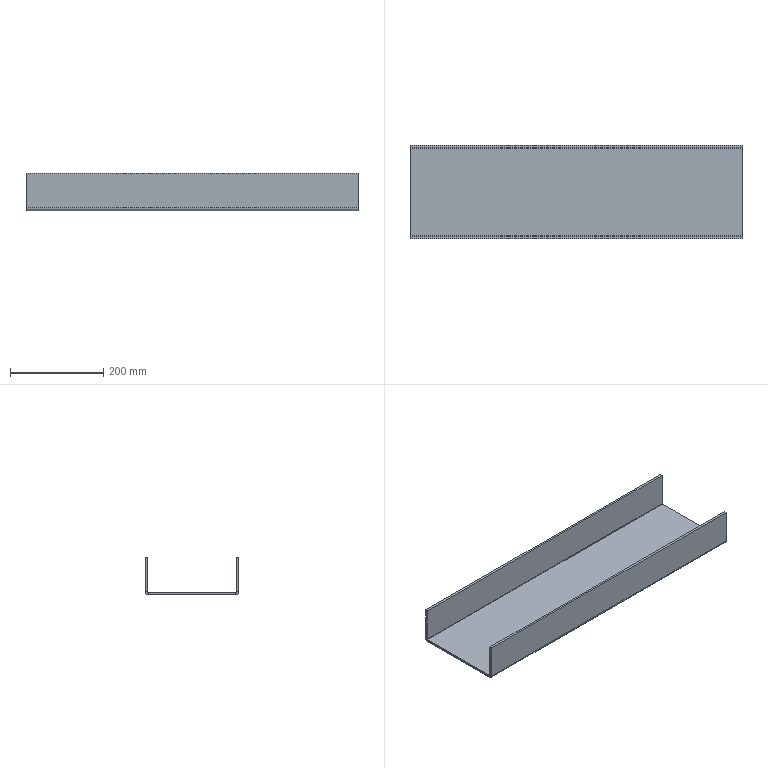Component | SolidWorks | ForkliftBasePlate-1 | 1 solid | 22 faces | box 712.5 x 200 x 80 mm | volume 1236977 mm3 | plane 18 | cylinder 4 | commonest cylinder face diameters 11.473 x2 1.473 x2 | material Q235
STEP:
#1=COLOUR_RGB('',0.7922,0.8196,0.9333);
#2=FILL_AREA_STYLE_COLOUR('',#1);
#3=FILL_AREA_STYLE('',(#2));
#4=SURFACE_STYLE_FILL_AREA(#3);
#5=SURFACE_SIDE_STYLE('',(#4));
#6=SURFACE_STYLE_USAGE(.BOTH.,#5);
#7=PRESENTATION_STYLE_ASSIGNMENT((#6));
#8=CARTESIAN_POINT('',(-18.136,36.701,107.705));
#9=VERTEX_POINT('',#8);
#10=CARTESIAN_POINT('',(-46.187,36.701,107.705));
#11=VERTEX_POINT('',#10);
#12=CARTESIAN_POINT('',(-18.136,36.701,107.705));
#13=DIRECTION('',(-1.,0.,0.));
#14=VECTOR('',#13,39.37);
#15=LINE('',#12,#14);
#16=EDGE_CURVE('',#9,#11,#15,.T.);
#17=ORIENTED_EDGE('',*,*,#16,.T.);
#18=CARTESIAN_POINT('',(-46.187,44.124,107.705));
#19=VERTEX_POINT('',#18);
#20=CARTESIAN_POINT('',(-46.187,44.349,107.705));
#21=DIRECTION('',(0.,-1.,0.));
#22=VECTOR('',#21,39.37);
#23=LINE('',#20,#22);
#24=EDGE_CURVE('',#19,#11,#23,.T.);
#25=ORIENTED_EDGE('',*,*,#24,.F.);
#26=CARTESIAN_POINT('',(-18.136,44.124,107.705));
#27=VERTEX_POINT('',#26);
#28=CARTESIAN_POINT('',(-46.187,44.124,107.705));
#29=DIRECTION('',(1.,0.,0.));
#30=VECTOR('',#29,39.37);
#31=LINE('',#28,#30);
#32=EDGE_CURVE('',#19,#27,#31,.T.);
#33=ORIENTED_EDGE('',*,*,#32,.T.);
#34=CARTESIAN_POINT('',(-18.136,44.349,107.705));
#35=DIRECTION('',(0.,1.,0.));
#36=VECTOR('',#35,39.37);
#37=LINE('',#34,#36);
#38=EDGE_CURVE('',#9,#27,#37,.T.);
#39=ORIENTED_EDGE('',*,*,#38,.F.);
#40=EDGE_LOOP('',(#17,#25,#33,#39));
#41=FACE_OUTER_BOUND('',#40,.T.);
#42=CARTESIAN_POINT('',(-32.162,40.412,107.705));
#43=DIRECTION('',(0.,0.,1.));
#44=DIRECTION('',(1.,0.,0.));
#45=AXIS2_PLACEMENT_3D('',#42,#43,#44);
#46=PLANE('',#45);
#47=ADVANCED_FACE('',(#41),#46,.F.);
#48=CARTESIAN_POINT('',(-46.187,44.124,107.902));
#49=VERTEX_POINT('',#48);
#50=CARTESIAN_POINT('',(-46.187,36.701,107.902));
#51=VERTEX_POINT('',#50);
#52=CARTESIAN_POINT('',(-46.187,44.349,107.902));
#53=DIRECTION('',(0.,-1.,0.));
#54=VECTOR('',#53,39.37);
#55=LINE('',#52,#54);
#56=EDGE_CURVE('',#49,#51,#55,.T.);
#57=ORIENTED_EDGE('',*,*,#56,.T.);
#58=CARTESIAN_POINT('',(-18.136,36.701,107.902));
#59=VERTEX_POINT('',#58);
#60=CARTESIAN_POINT('',(-18.136,36.701,107.902));
#61=DIRECTION('',(-1.,0.,0.));
#62=VECTOR('',#61,39.37);
#63=LINE('',#60,#62);
#64=EDGE_CURVE('',#59,#51,#63,.T.);
#65=ORIENTED_EDGE('',*,*,#64,.F.);
#66=CARTESIAN_POINT('',(-18.136,44.124,107.902));
#67=VERTEX_POINT('',#66);
#68=CARTESIAN_POINT('',(-18.136,44.349,107.902));
#69=DIRECTION('',(0.,1.,0.));
#70=VECTOR('',#69,39.37);
#71=LINE('',#68,#70);
#72=EDGE_CURVE('',#59,#67,#71,.T.);
#73=ORIENTED_EDGE('',*,*,#72,.T.);
#74=CARTESIAN_POINT('',(-46.187,44.124,107.902));
#75=DIRECTION('',(1.,0.,0.));
#76=VECTOR('',#75,39.37);
#77=LINE('',#74,#76);
#78=EDGE_CURVE('',#49,#67,#77,.T.);
#79=ORIENTED_EDGE('',*,*,#78,.F.);
#80=EDGE_LOOP('',(#57,#65,#73,#79));
#81=FACE_OUTER_BOUND('',#80,.T.);
#82=CARTESIAN_POINT('',(-32.162,40.412,107.902));
#83=DIRECTION('',(0.,0.,1.));
#84=DIRECTION('',(1.,0.,0.));
#85=AXIS2_PLACEMENT_3D('',#82,#83,#84);
#86=PLANE('',#85);
#87=ADVANCED_FACE('',(#81),#86,.T.);
#88=ORIENTED_EDGE('',*,*,#72,.F.);
#89=CARTESIAN_POINT('',(-18.136,36.701,107.902));
#90=DIRECTION('',(0.,0.,-1.));
#91=VECTOR('',#90,39.37);
#92=LINE('',#89,#91);
#93=EDGE_CURVE('',#59,#9,#92,.T.);
#94=ORIENTED_EDGE('',*,*,#93,.T.);
#95=ORIENTED_EDGE('',*,*,#38,.T.);
#96=CARTESIAN_POINT('',(-18.136,44.124,107.902));
#97=DIRECTION('',(0.,0.,-1.));
#98=VECTOR('',#97,39.37);
#99=LINE('',#96,#98);
#100=EDGE_CURVE('',#67,#27,#99,.T.);
#101=ORIENTED_EDGE('',*,*,#100,.F.);
#102=EDGE_LOOP('',(#88,#94,#95,#101));
#103=FACE_OUTER_BOUND('',#102,.T.);
#104=CARTESIAN_POINT('',(-18.136,44.349,107.705));
#105=DIRECTION('',(1.,0.,0.));
#106=DIRECTION('',(0.,0.,-1.));
#107=AXIS2_PLACEMENT_3D('',#104,#105,#106);
#108=PLANE('',#107);
#109=ADVANCED_FACE('',(#103),#108,.T.);
#110=CARTESIAN_POINT('',(-46.187,36.701,107.902));
#111=DIRECTION('',(0.,0.,-1.));
#112=VECTOR('',#111,39.37);
#113=LINE('',#110,#112);
#114=EDGE_CURVE('',#51,#11,#113,.T.);
#115=ORIENTED_EDGE('',*,*,#114,.F.);
#116=ORIENTED_EDGE('',*,*,#56,.F.);
#117=CARTESIAN_POINT('',(-46.187,44.124,107.902));
#118=DIRECTION('',(0.,0.,-1.));
#119=VECTOR('',#118,39.37);
#120=LINE('',#117,#119);
#121=EDGE_CURVE('',#49,#19,#120,.T.);
#122=ORIENTED_EDGE('',*,*,#121,.T.);
#123=ORIENTED_EDGE('',*,*,#24,.T.);
#124=EDGE_LOOP('',(#115,#116,#122,#123));
#125=FACE_OUTER_BOUND('',#124,.T.);
#126=CARTESIAN_POINT('',(-46.187,44.349,107.705));
#127=DIRECTION('',(-1.,0.,0.));
#128=DIRECTION('',(0.,0.,1.));
#129=AXIS2_PLACEMENT_3D('',#126,#127,#128);
#130=PLANE('',#129);
#131=ADVANCED_FACE('',(#125),#130,.T.);
#132=CARTESIAN_POINT('',(-18.136,44.153,107.931));
#133=VERTEX_POINT('',#132);
#134=CARTESIAN_POINT('',(-18.136,44.349,107.931));
#135=VERTEX_POINT('',#134);
#136=CARTESIAN_POINT('',(-18.136,44.349,107.931));
#137=DIRECTION('',(0.,1.,-0.));
#138=VECTOR('',#137,39.37);
#139=LINE('',#136,#138);
#140=EDGE_CURVE('',#133,#135,#139,.T.);
#141=ORIENTED_EDGE('',*,*,#140,.F.);
#142=CARTESIAN_POINT('',(-18.136,44.124,107.931));
#143=DIRECTION('',(1.,0.,0.));
#144=DIRECTION('',(0.,0.,1.));
#145=AXIS2_PLACEMENT_3D('',#142,#143,#144);
#146=CIRCLE('',#145,0.029);
#147=EDGE_CURVE('',#67,#133,#146,.T.);
#148=ORIENTED_EDGE('',*,*,#147,.F.);
#149=ORIENTED_EDGE('',*,*,#100,.T.);
#150=CARTESIAN_POINT('',(-18.136,44.124,107.931));
#151=DIRECTION('',(1.,0.,0.));
#152=DIRECTION('',(0.,0.,1.));
#153=AXIS2_PLACEMENT_3D('',#150,#151,#152);
#154=CIRCLE('',#153,0.2259);
#155=EDGE_CURVE('',#27,#135,#154,.T.);
#156=ORIENTED_EDGE('',*,*,#155,.T.);
#157=EDGE_LOOP('',(#141,#148,#149,#156));
#158=FACE_OUTER_BOUND('',#157,.T.);
#159=CARTESIAN_POINT('',(-18.136,44.124,107.931));
#160=DIRECTION('',(1.,0.,0.));
#161=DIRECTION('',(0.,0.,-1.));
#162=AXIS2_PLACEMENT_3D('',#159,#160,#161);
#163=PLANE('',#162);
#164=ADVANCED_FACE('',(#158),#163,.T.);
#165=CARTESIAN_POINT('',(-46.187,44.153,107.931));
#166=VERTEX_POINT('',#165);
#167=CARTESIAN_POINT('',(-46.187,44.124,107.931));
#168=DIRECTION('',(-1.,0.,0.));
#169=DIRECTION('',(0.,0.,1.));
#170=AXIS2_PLACEMENT_3D('',#167,#168,#169);
#171=CIRCLE('',#170,0.029);
#172=EDGE_CURVE('',#166,#49,#171,.T.);
#173=ORIENTED_EDGE('',*,*,#172,.F.);
#174=CARTESIAN_POINT('',(-46.187,44.349,107.931));
#175=VERTEX_POINT('',#174);
#176=CARTESIAN_POINT('',(-46.187,44.153,107.931));
#177=DIRECTION('',(0.,1.,-0.));
#178=VECTOR('',#177,39.37);
#179=LINE('',#176,#178);
#180=EDGE_CURVE('',#166,#175,#179,.T.);
#181=ORIENTED_EDGE('',*,*,#180,.T.);
#182=CARTESIAN_POINT('',(-46.187,44.124,107.931));
#183=DIRECTION('',(-1.,0.,0.));
#184=DIRECTION('',(0.,0.,1.));
#185=AXIS2_PLACEMENT_3D('',#182,#183,#184);
#186=CIRCLE('',#185,0.2259);
#187=EDGE_CURVE('',#175,#19,#186,.T.);
#188=ORIENTED_EDGE('',*,*,#187,.T.);
#189=ORIENTED_EDGE('',*,*,#121,.F.);
#190=EDGE_LOOP('',(#173,#181,#188,#189));
#191=FACE_OUTER_BOUND('',#190,.T.);
#192=CARTESIAN_POINT('',(-46.187,44.124,107.931));
#193=DIRECTION('',(1.,0.,0.));
#194=DIRECTION('',(0.,0.,-1.));
#195=AXIS2_PLACEMENT_3D('',#192,#193,#194);
#196=PLANE('',#195);
#197=ADVANCED_FACE('',(#191),#196,.F.);
#198=ORIENTED_EDGE('',*,*,#32,.F.);
#199=ORIENTED_EDGE('',*,*,#187,.F.);
#200=CARTESIAN_POINT('',(-32.162,44.349,107.931));
#201=DIRECTION('',(-1.,-0.,-0.));
#202=VECTOR('',#201,39.37);
#203=LINE('',#200,#202);
#204=EDGE_CURVE('',#135,#175,#203,.T.);
#205=ORIENTED_EDGE('',*,*,#204,.F.);
#206=ORIENTED_EDGE('',*,*,#155,.F.);
#207=EDGE_LOOP('',(#198,#199,#205,#206));
#208=FACE_OUTER_BOUND('',#207,.T.);
#209=CARTESIAN_POINT('',(-46.187,44.124,107.931));
#210=DIRECTION('',(-1.,0.,0.));
#211=DIRECTION('',(0.,1.,0.));
#212=AXIS2_PLACEMENT_3D('',#209,#210,#211);
#213=CYLINDRICAL_SURFACE('',#212,0.2259);
#214=ADVANCED_FACE('',(#208),#213,.T.);
#215=ORIENTED_EDGE('',*,*,#78,.T.);
#216=ORIENTED_EDGE('',*,*,#147,.T.);
#217=CARTESIAN_POINT('',(-18.136,44.153,107.931));
#218=DIRECTION('',(-1.,-0.,-0.));
#219=VECTOR('',#218,39.37);
#220=LINE('',#217,#219);
#221=EDGE_CURVE('',#133,#166,#220,.T.);
#222=ORIENTED_EDGE('',*,*,#221,.T.);
#223=ORIENTED_EDGE('',*,*,#172,.T.);
#224=EDGE_LOOP('',(#215,#216,#222,#223));
#225=FACE_OUTER_BOUND('',#224,.T.);
#226=CARTESIAN_POINT('',(-46.187,44.124,107.931));
#227=DIRECTION('',(-1.,0.,0.));
#228=DIRECTION('',(0.,1.,0.));
#229=AXIS2_PLACEMENT_3D('',#226,#227,#228);
#230=CYLINDRICAL_SURFACE('',#229,0.029);
#231=ADVANCED_FACE('',(#225),#230,.F.);
#232=CARTESIAN_POINT('',(-46.187,44.349,110.855));
#233=VERTEX_POINT('',#232);
#234=CARTESIAN_POINT('',(-46.187,44.349,107.902));
#235=DIRECTION('',(0.,-0.,-1.));
#236=VECTOR('',#235,39.37);
#237=LINE('',#234,#236);
#238=EDGE_CURVE('',#233,#175,#237,.T.);
#239=ORIENTED_EDGE('',*,*,#238,.T.);
#240=ORIENTED_EDGE('',*,*,#180,.F.);
#241=CARTESIAN_POINT('',(-46.187,44.153,110.855));
#242=VERTEX_POINT('',#241);
#243=CARTESIAN_POINT('',(-46.187,44.153,107.902));
#244=DIRECTION('',(0.,-0.,-1.));
#245=VECTOR('',#244,39.37);
#246=LINE('',#243,#245);
#247=EDGE_CURVE('',#242,#166,#246,.T.);
#248=ORIENTED_EDGE('',*,*,#247,.F.);
#249=CARTESIAN_POINT('',(-46.187,44.349,110.855));
#250=DIRECTION('',(0.,-1.,0.));
#251=VECTOR('',#250,39.37);
#252=LINE('',#249,#251);
#253=EDGE_CURVE('',#233,#242,#252,.T.);
#254=ORIENTED_EDGE('',*,*,#253,.F.);
#255=EDGE_LOOP('',(#239,#240,#248,#254));
#256=FACE_OUTER_BOUND('',#255,.T.);
#257=CARTESIAN_POINT('',(-46.187,44.349,107.902));
#258=DIRECTION('',(-1.,0.,0.));
#259=DIRECTION('',(0.,0.,1.));
#260=AXIS2_PLACEMENT_3D('',#257,#258,#259);
#261=PLANE('',#260);
#262=ADVANCED_FACE('',(#256),#261,.T.);
#263=CARTESIAN_POINT('',(-18.136,44.153,110.855));
#264=VERTEX_POINT('',#263);
#265=CARTESIAN_POINT('',(-18.136,44.153,107.902));
#266=DIRECTION('',(0.,0.,1.));
#267=VECTOR('',#266,39.37);
#268=LINE('',#265,#267);
#269=EDGE_CURVE('',#133,#264,#268,.T.);
#270=ORIENTED_EDGE('',*,*,#269,.F.);
#271=ORIENTED_EDGE('',*,*,#140,.T.);
#272=CARTESIAN_POINT('',(-18.136,44.349,110.855));
#273=VERTEX_POINT('',#272);
#274=CARTESIAN_POINT('',(-18.136,44.349,110.855));
#275=DIRECTION('',(0.,0.,1.));
#276=VECTOR('',#275,39.37);
#277=LINE('',#274,#276);
#278=EDGE_CURVE('',#135,#273,#277,.T.);
#279=ORIENTED_EDGE('',*,*,#278,.T.);
#280=CARTESIAN_POINT('',(-18.136,44.349,110.855));
#281=DIRECTION('',(0.,-1.,0.));
#282=VECTOR('',#281,39.37);
#283=LINE('',#280,#282);
#284=EDGE_CURVE('',#273,#264,#283,.T.);
#285=ORIENTED_EDGE('',*,*,#284,.T.);
#286=EDGE_LOOP('',(#270,#271,#279,#285));
#287=FACE_OUTER_BOUND('',#286,.T.);
#288=CARTESIAN_POINT('',(-18.136,44.349,110.855));
#289=DIRECTION('',(1.,0.,0.));
#290=DIRECTION('',(0.,0.,-1.));
#291=AXIS2_PLACEMENT_3D('',#288,#289,#290);
#292=PLANE('',#291);
#293=ADVANCED_FACE('',(#287),#292,.T.);
#294=ORIENTED_EDGE('',*,*,#278,.F.);
#295=ORIENTED_EDGE('',*,*,#204,.T.);
#296=ORIENTED_EDGE('',*,*,#238,.F.);
#297=CARTESIAN_POINT('',(-46.187,44.349,110.855));
#298=DIRECTION('',(-1.,0.,0.));
#299=VECTOR('',#298,39.37);
#300=LINE('',#297,#299);
#301=EDGE_CURVE('',#273,#233,#300,.T.);
#302=ORIENTED_EDGE('',*,*,#301,.F.);
#303=EDGE_LOOP('',(#294,#295,#296,#302));
#304=FACE_OUTER_BOUND('',#303,.T.);
#305=CARTESIAN_POINT('',(-32.162,44.349,107.902));
#306=DIRECTION('',(0.,1.,-0.));
#307=DIRECTION('',(0.,0.,1.));
#308=AXIS2_PLACEMENT_3D('',#305,#306,#307);
#309=PLANE('',#308);
#310=ADVANCED_FACE('',(#304),#309,.T.);
#311=ORIENTED_EDGE('',*,*,#221,.F.);
#312=ORIENTED_EDGE('',*,*,#269,.T.);
#313=CARTESIAN_POINT('',(-32.162,44.153,110.855));
#314=DIRECTION('',(-1.,0.,0.));
#315=VECTOR('',#314,39.37);
#316=LINE('',#313,#315);
#317=EDGE_CURVE('',#264,#242,#316,.T.);
#318=ORIENTED_EDGE('',*,*,#317,.T.);
#319=ORIENTED_EDGE('',*,*,#247,.T.);
#320=EDGE_LOOP('',(#311,#312,#318,#319));
#321=FACE_OUTER_BOUND('',#320,.T.);
#322=CARTESIAN_POINT('',(-32.162,44.153,107.902));
#323=DIRECTION('',(0.,1.,-0.));
#324=DIRECTION('',(0.,0.,1.));
#325=AXIS2_PLACEMENT_3D('',#322,#323,#324);
#326=PLANE('',#325);
#327=ADVANCED_FACE('',(#321),#326,.F.);
#328=ORIENTED_EDGE('',*,*,#317,.F.);
#329=ORIENTED_EDGE('',*,*,#284,.F.);
#330=ORIENTED_EDGE('',*,*,#301,.T.);
#331=ORIENTED_EDGE('',*,*,#253,.T.);
#332=EDGE_LOOP('',(#328,#329,#330,#331));
#333=FACE_OUTER_BOUND('',#332,.T.);
#334=CARTESIAN_POINT('',(-46.187,44.349,110.855));
#335=DIRECTION('',(0.,0.,1.));
#336=DIRECTION('',(0.,-1.,0.));
#337=AXIS2_PLACEMENT_3D('',#334,#335,#336);
#338=PLANE('',#337);
#339=ADVANCED_FACE('',(#333),#338,.T.);
#340=CARTESIAN_POINT('',(-46.187,36.672,107.931));
#341=VERTEX_POINT('',#340);
#342=CARTESIAN_POINT('',(-46.187,36.475,107.931));
#343=VERTEX_POINT('',#342);
#344=CARTESIAN_POINT('',(-46.187,36.475,107.931));
#345=DIRECTION('',(0.,-1.,-0.));
#346=VECTOR('',#345,39.37);
#347=LINE('',#344,#346);
#348=EDGE_CURVE('',#341,#343,#347,.T.);
#349=ORIENTED_EDGE('',*,*,#348,.F.);
#350=CARTESIAN_POINT('',(-46.187,36.701,107.931));
#351=DIRECTION('',(-1.,0.,0.));
#352=DIRECTION('',(0.,0.,-1.));
#353=AXIS2_PLACEMENT_3D('',#350,#351,#352);
#354=CIRCLE('',#353,0.029);
#355=EDGE_CURVE('',#51,#341,#354,.T.);
#356=ORIENTED_EDGE('',*,*,#355,.F.);
#357=ORIENTED_EDGE('',*,*,#114,.T.);
#358=CARTESIAN_POINT('',(-46.187,36.701,107.931));
#359=DIRECTION('',(-1.,0.,0.));
#360=DIRECTION('',(0.,0.,-1.));
#361=AXIS2_PLACEMENT_3D('',#358,#359,#360);
#362=CIRCLE('',#361,0.2259);
#363=EDGE_CURVE('',#11,#343,#362,.T.);
#364=ORIENTED_EDGE('',*,*,#363,.T.);
#365=EDGE_LOOP('',(#349,#356,#357,#364));
#366=FACE_OUTER_BOUND('',#365,.T.);
#367=CARTESIAN_POINT('',(-46.187,36.701,107.931));
#368=DIRECTION('',(-1.,0.,0.));
#369=DIRECTION('',(0.,0.,1.));
#370=AXIS2_PLACEMENT_3D('',#367,#368,#369);
#371=PLANE('',#370);
#372=ADVANCED_FACE('',(#366),#371,.T.);
#373=CARTESIAN_POINT('',(-18.136,36.672,107.931));
#374=VERTEX_POINT('',#373);
#375=CARTESIAN_POINT('',(-18.136,36.701,107.931));
#376=DIRECTION('',(1.,0.,0.));
#377=DIRECTION('',(0.,0.,-1.));
#378=AXIS2_PLACEMENT_3D('',#375,#376,#377);
#379=CIRCLE('',#378,0.029);
#380=EDGE_CURVE('',#374,#59,#379,.T.);
#381=ORIENTED_EDGE('',*,*,#380,.F.);
#382=CARTESIAN_POINT('',(-18.136,36.475,107.931));
#383=VERTEX_POINT('',#382);
#384=CARTESIAN_POINT('',(-18.136,36.672,107.931));
#385=DIRECTION('',(0.,-1.,-0.));
#386=VECTOR('',#385,39.37);
#387=LINE('',#384,#386);
#388=EDGE_CURVE('',#374,#383,#387,.T.);
#389=ORIENTED_EDGE('',*,*,#388,.T.);
#390=CARTESIAN_POINT('',(-18.136,36.701,107.931));
#391=DIRECTION('',(1.,0.,0.));
#392=DIRECTION('',(0.,0.,-1.));
#393=AXIS2_PLACEMENT_3D('',#390,#391,#392);
#394=CIRCLE('',#393,0.2259);
#395=EDGE_CURVE('',#383,#9,#394,.T.);
#396=ORIENTED_EDGE('',*,*,#395,.T.);
#397=ORIENTED_EDGE('',*,*,#93,.F.);
#398=EDGE_LOOP('',(#381,#389,#396,#397));
#399=FACE_OUTER_BOUND('',#398,.T.);
#400=CARTESIAN_POINT('',(-18.136,36.701,107.931));
#401=DIRECTION('',(-1.,0.,0.));
#402=DIRECTION('',(0.,0.,1.));
#403=AXIS2_PLACEMENT_3D('',#400,#401,#402);
#404=PLANE('',#403);
#405=ADVANCED_FACE('',(#399),#404,.F.);
#406=ORIENTED_EDGE('',*,*,#16,.F.);
#407=ORIENTED_EDGE('',*,*,#395,.F.);
#408=CARTESIAN_POINT('',(-32.162,36.475,107.931));
#409=DIRECTION('',(1.,-0.,0.));
#410=VECTOR('',#409,39.37);
#411=LINE('',#408,#410);
#412=EDGE_CURVE('',#343,#383,#411,.T.);
#413=ORIENTED_EDGE('',*,*,#412,.F.);
#414=ORIENTED_EDGE('',*,*,#363,.F.);
#415=EDGE_LOOP('',(#406,#407,#413,#414));
#416=FACE_OUTER_BOUND('',#415,.T.);
#417=CARTESIAN_POINT('',(-18.136,36.701,107.931));
#418=DIRECTION('',(1.,0.,0.));
#419=DIRECTION('',(0.,-1.,0.));
#420=AXIS2_PLACEMENT_3D('',#417,#418,#419);
#421=CYLINDRICAL_SURFACE('',#420,0.2259);
#422=ADVANCED_FACE('',(#416),#421,.T.);
#423=ORIENTED_EDGE('',*,*,#64,.T.);
#424=ORIENTED_EDGE('',*,*,#355,.T.);
#425=CARTESIAN_POINT('',(-46.187,36.672,107.931));
#426=DIRECTION('',(1.,-0.,0.));
#427=VECTOR('',#426,39.37);
#428=LINE('',#425,#427);
#429=EDGE_CURVE('',#341,#374,#428,.T.);
#430=ORIENTED_EDGE('',*,*,#429,.T.);
#431=ORIENTED_EDGE('',*,*,#380,.T.);
#432=EDGE_LOOP('',(#423,#424,#430,#431));
#433=FACE_OUTER_BOUND('',#432,.T.);
#434=CARTESIAN_POINT('',(-18.136,36.701,107.931));
#435=DIRECTION('',(1.,0.,0.));
#436=DIRECTION('',(0.,-1.,0.));
#437=AXIS2_PLACEMENT_3D('',#434,#435,#436);
#438=CYLINDRICAL_SURFACE('',#437,0.029);
#439=ADVANCED_FACE('',(#433),#438,.F.);
#440=CARTESIAN_POINT('',(-18.136,36.475,110.855));
#441=VERTEX_POINT('',#440);
#442=CARTESIAN_POINT('',(-18.136,36.475,107.902));
#443=DIRECTION('',(0.,0.,-1.));
#444=VECTOR('',#443,39.37);
#445=LINE('',#442,#444);
#446=EDGE_CURVE('',#441,#383,#445,.T.);
#447=ORIENTED_EDGE('',*,*,#446,.T.);
#448=ORIENTED_EDGE('',*,*,#388,.F.);
#449=CARTESIAN_POINT('',(-18.136,36.672,110.855));
#450=VERTEX_POINT('',#449);
#451=CARTESIAN_POINT('',(-18.136,36.672,107.902));
#452=DIRECTION('',(0.,0.,-1.));
#453=VECTOR('',#452,39.37);
#454=LINE('',#451,#453);
#455=EDGE_CURVE('',#450,#374,#454,.T.);
#456=ORIENTED_EDGE('',*,*,#455,.F.);
#457=CARTESIAN_POINT('',(-18.136,36.475,110.855));
#458=DIRECTION('',(0.,1.,0.));
#459=VECTOR('',#458,39.37);
#460=LINE('',#457,#459);
#461=EDGE_CURVE('',#441,#450,#460,.T.);
#462=ORIENTED_EDGE('',*,*,#461,.F.);
#463=EDGE_LOOP('',(#447,#448,#456,#462));
#464=FACE_OUTER_BOUND('',#463,.T.);
#465=CARTESIAN_POINT('',(-18.136,36.475,107.902));
#466=DIRECTION('',(1.,0.,0.));
#467=DIRECTION('',(0.,0.,-1.));
#468=AXIS2_PLACEMENT_3D('',#465,#466,#467);
#469=PLANE('',#468);
#470=ADVANCED_FACE('',(#464),#469,.T.);
#471=CARTESIAN_POINT('',(-46.187,36.672,110.855));
#472=VERTEX_POINT('',#471);
#473=CARTESIAN_POINT('',(-46.187,36.672,107.902));
#474=DIRECTION('',(0.,-0.,1.));
#475=VECTOR('',#474,39.37);
#476=LINE('',#473,#475);
#477=EDGE_CURVE('',#341,#472,#476,.T.);
#478=ORIENTED_EDGE('',*,*,#477,.F.);
#479=ORIENTED_EDGE('',*,*,#348,.T.);
#480=CARTESIAN_POINT('',(-46.187,36.475,110.855));
#481=VERTEX_POINT('',#480);
#482=CARTESIAN_POINT('',(-46.187,36.475,110.855));
#483=DIRECTION('',(0.,-0.,1.));
#484=VECTOR('',#483,39.37);
#485=LINE('',#482,#484);
#486=EDGE_CURVE('',#343,#481,#485,.T.);
#487=ORIENTED_EDGE('',*,*,#486,.T.);
#488=CARTESIAN_POINT('',(-46.187,36.475,110.855));
#489=DIRECTION('',(0.,1.,0.));
#490=VECTOR('',#489,39.37);
#491=LINE('',#488,#490);
#492=EDGE_CURVE('',#481,#472,#491,.T.);
#493=ORIENTED_EDGE('',*,*,#492,.T.);
#494=EDGE_LOOP('',(#478,#479,#487,#493));
#495=FACE_OUTER_BOUND('',#494,.T.);
#496=CARTESIAN_POINT('',(-46.187,36.475,110.855));
#497=DIRECTION('',(-1.,0.,0.));
#498=DIRECTION('',(0.,0.,1.));
#499=AXIS2_PLACEMENT_3D('',#496,#497,#498);
#500=PLANE('',#499);
#501=ADVANCED_FACE('',(#495),#500,.T.);
#502=ORIENTED_EDGE('',*,*,#486,.F.);
#503=ORIENTED_EDGE('',*,*,#412,.T.);
#504=ORIENTED_EDGE('',*,*,#446,.F.);
#505=CARTESIAN_POINT('',(-18.136,36.475,110.855));
#506=DIRECTION('',(1.,0.,0.));
#507=VECTOR('',#506,39.37);
#508=LINE('',#505,#507);
#509=EDGE_CURVE('',#481,#441,#508,.T.);
#510=ORIENTED_EDGE('',*,*,#509,.F.);
#511=EDGE_LOOP('',(#502,#503,#504,#510));
#512=FACE_OUTER_BOUND('',#511,.T.);
#513=CARTESIAN_POINT('',(-32.162,36.475,107.902));
#514=DIRECTION('',(0.,-1.,-0.));
#515=DIRECTION('',(0.,0.,-1.));
#516=AXIS2_PLACEMENT_3D('',#513,#514,#515);
#517=PLANE('',#516);
#518=ADVANCED_FACE('',(#512),#517,.T.);
#519=ORIENTED_EDGE('',*,*,#429,.F.);
#520=ORIENTED_EDGE('',*,*,#477,.T.);
#521=CARTESIAN_POINT('',(-32.162,36.672,110.855));
#522=DIRECTION('',(1.,0.,0.));
#523=VECTOR('',#522,39.37);
#524=LINE('',#521,#523);
#525=EDGE_CURVE('',#472,#450,#524,.T.);
#526=ORIENTED_EDGE('',*,*,#525,.T.);
#527=ORIENTED_EDGE('',*,*,#455,.T.);
#528=EDGE_LOOP('',(#519,#520,#526,#527));
#529=FACE_OUTER_BOUND('',#528,.T.);
#530=CARTESIAN_POINT('',(-32.162,36.672,107.902));
#531=DIRECTION('',(0.,-1.,-0.));
#532=DIRECTION('',(0.,0.,-1.));
#533=AXIS2_PLACEMENT_3D('',#530,#531,#532);
#534=PLANE('',#533);
#535=ADVANCED_FACE('',(#529),#534,.F.);
#536=ORIENTED_EDGE('',*,*,#525,.F.);
#537=ORIENTED_EDGE('',*,*,#492,.F.);
#538=ORIENTED_EDGE('',*,*,#509,.T.);
#539=ORIENTED_EDGE('',*,*,#461,.T.);
#540=EDGE_LOOP('',(#536,#537,#538,#539));
#541=FACE_OUTER_BOUND('',#540,.T.);
#542=CARTESIAN_POINT('',(-18.136,36.475,110.855));
#543=DIRECTION('',(0.,-0.,1.));
#544=DIRECTION('',(0.,-1.,-0.));
#545=AXIS2_PLACEMENT_3D('',#542,#543,#544);
#546=PLANE('',#545);
#547=ADVANCED_FACE('',(#541),#546,.T.);
#548=CLOSED_SHELL('',(#47,#87,#109,#131,#164,#197,#214,#231,#262,#293,#310,#327,#339,#372,#405,#422,#439,#470,#501,#518,#535,#547));
#549=MANIFOLD_SOLID_BREP('',#548);
#550=STYLED_ITEM('',(#7),#549);
#551=(LENGTH_UNIT()NAMED_UNIT(*)SI_UNIT($,.METRE.));
#552=LENGTH_MEASURE_WITH_UNIT(LENGTH_MEASURE(0.0254),#551);
#553=DIMENSIONAL_EXPONENTS(1.,0.,0.,0.,0.,0.,0.);
#554=(CONVERSION_BASED_UNIT('',#552)LENGTH_UNIT()NAMED_UNIT(#553));
#555=UNCERTAINTY_MEASURE_WITH_UNIT(LENGTH_MEASURE(0.00001),#554,'','');
#556=(NAMED_UNIT(*)PLANE_ANGLE_UNIT()SI_UNIT($,.RADIAN.));
#557=(NAMED_UNIT(*)SI_UNIT($,.STERADIAN.)SOLID_ANGLE_UNIT());
#558=(GEOMETRIC_REPRESENTATION_CONTEXT(3)GLOBAL_UNCERTAINTY_ASSIGNED_CONTEXT((#555))GLOBAL_UNIT_ASSIGNED_CONTEXT((#554,#556,#557))REPRESENTATION_CONTEXT('',''));
#559=MECHANICAL_DESIGN_GEOMETRIC_PRESENTATION_REPRESENTATION('',(#550),#558);
#560=PRESENTATION_LAYER_ASSIGNMENT('','',(#550));
#561=CARTESIAN_POINT('',(0.,0.,0.));
#562=DIRECTION('',(0.,0.,1.));
#563=DIRECTION('',(1.,0.,0.));
#564=AXIS2_PLACEMENT_3D('',#561,#562,#563);
#565=(LENGTH_UNIT()NAMED_UNIT(*)SI_UNIT($,.METRE.));
#566=LENGTH_MEASURE_WITH_UNIT(LENGTH_MEASURE(0.0254),#565);
#567=DIMENSIONAL_EXPONENTS(1.,0.,0.,0.,0.,0.,0.);
#568=(CONVERSION_BASED_UNIT('',#566)LENGTH_UNIT()NAMED_UNIT(#567));
#569=UNCERTAINTY_MEASURE_WITH_UNIT(LENGTH_MEASURE(0.00001),#568,'','');
#570=(NAMED_UNIT(*)PLANE_ANGLE_UNIT()SI_UNIT($,.RADIAN.));
#571=(NAMED_UNIT(*)SI_UNIT($,.STERADIAN.)SOLID_ANGLE_UNIT());
#572=(GEOMETRIC_REPRESENTATION_CONTEXT(3)GLOBAL_UNCERTAINTY_ASSIGNED_CONTEXT((#569))GLOBAL_UNIT_ASSIGNED_CONTEXT((#568,#570,#571))REPRESENTATION_CONTEXT('',''));
#573=ADVANCED_BREP_SHAPE_REPRESENTATION('',(#549,#564),#572);